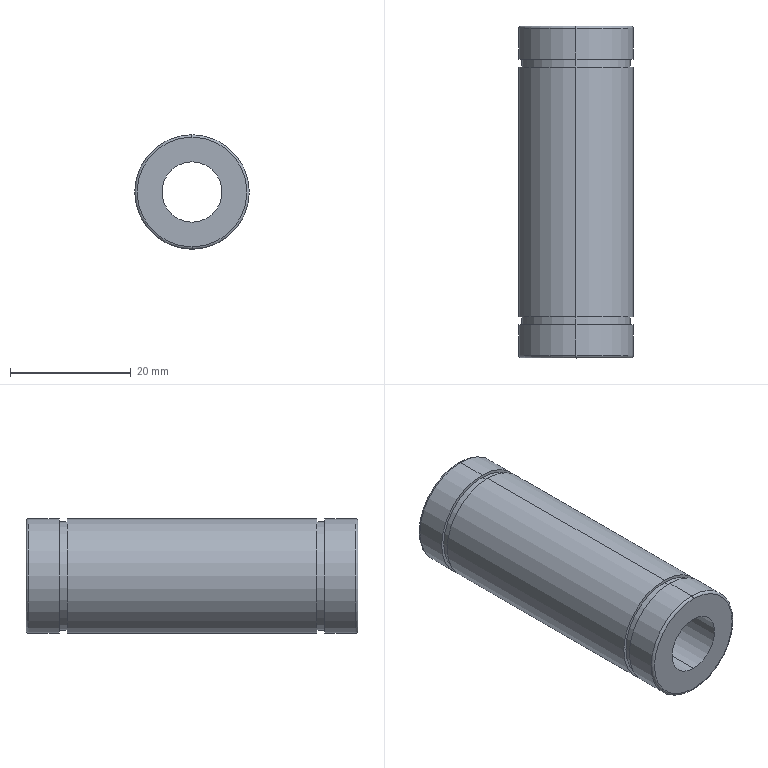Component | SolidWorks | LMUW10-3 | 1 solid | 22 faces | box 19 x 55 x 19 mm | volume 11195 mm3 | cylinder 12 | plane 6 | torus 4 | commonest cylinder face diameters 19 x6 18 x4 10 x2
build123d program:
from build123d import *


with BuildPart() as part:
    # Sketch1 → Revolve1 (revolve)
    with BuildSketch(Plane.XY, mode=Mode.PRIVATE) as revolve1_sk:
        with BuildLine():
            Line((0, 9.1), (0, 5))
            Line((0, 5), (55, 5))
            Line((55, 5), (55, 9.1))
            ThreePointArc((55, 9.1), (54.883, 9.383), (54.6, 9.5))
            Line((54.6, 9.5), (49.5, 9.5))
            Line((49.5, 9.5), (49.5, 9))
            Line((49.5, 9), (48.2, 9))
            Line((48.2, 9), (48.2, 9.5))
            Line((48.2, 9.5), (6.8, 9.5))
            Line((6.8, 9.5), (6.8, 9))
            Line((6.8, 9), (5.5, 9))
            Line((5.5, 9), (5.5, 9.5))
            Line((5.5, 9.5), (0.4, 9.5))
            ThreePointArc((0.4, 9.5), (0.1172, 9.383), (0, 9.1))
        make_face()
    revolve(revolve1_sk.sketch.rotate(Axis((27.5, 0, 0), (-1, 0, 0)), 270), axis=Axis((27.5, 0, 0), (-1, 0, 0)))


solid = part.part

# Placed as in the assembly
solid = solid.moved(Location((294.5, -645.807, -22.94), (0, 0, 90)))
STEP:
#1=COLOUR_RGB('',0.7922,0.8196,0.9333);
#2=FILL_AREA_STYLE_COLOUR('',#1);
#3=FILL_AREA_STYLE('',(#2));
#4=SURFACE_STYLE_FILL_AREA(#3);
#5=SURFACE_SIDE_STYLE('',(#4));
#6=SURFACE_STYLE_USAGE(.BOTH.,#5);
#7=PRESENTATION_STYLE_ASSIGNMENT((#6));
#8=CARTESIAN_POINT('',(11.594,-25.209,-0.5292));
#9=VERTEX_POINT('',#8);
#10=CARTESIAN_POINT('',(11.594,-25.209,-1.277));
#11=VERTEX_POINT('',#10);
#12=CARTESIAN_POINT('',(11.594,-25.209,-0.9032));
#13=DIRECTION('',(0.,-1.,-0.));
#14=DIRECTION('',(-0.,0.,1.));
#15=AXIS2_PLACEMENT_3D('',#12,#13,#14);
#16=CIRCLE('',#15,0.374);
#17=EDGE_CURVE('',#9,#11,#16,.T.);
#18=ORIENTED_EDGE('',*,*,#17,.T.);
#19=CARTESIAN_POINT('',(11.594,-25.41,-1.277));
#20=VERTEX_POINT('',#19);
#21=CARTESIAN_POINT('',(11.594,-24.343,-1.277));
#22=DIRECTION('',(0.,-1.,-0.));
#23=VECTOR('',#22,39.37);
#24=LINE('',#21,#23);
#25=EDGE_CURVE('',#11,#20,#24,.T.);
#26=ORIENTED_EDGE('',*,*,#25,.T.);
#27=CARTESIAN_POINT('',(11.594,-25.41,-0.5292));
#28=VERTEX_POINT('',#27);
#29=CARTESIAN_POINT('',(11.594,-25.41,-0.9032));
#30=DIRECTION('',(0.,-1.,-0.));
#31=DIRECTION('',(-0.,0.,1.));
#32=AXIS2_PLACEMENT_3D('',#29,#30,#31);
#33=CIRCLE('',#32,0.374);
#34=EDGE_CURVE('',#28,#20,#33,.T.);
#35=ORIENTED_EDGE('',*,*,#34,.F.);
#36=CARTESIAN_POINT('',(11.594,-24.343,-0.5292));
#37=DIRECTION('',(0.,-1.,-0.));
#38=VECTOR('',#37,39.37);
#39=LINE('',#36,#38);
#40=EDGE_CURVE('',#9,#28,#39,.T.);
#41=ORIENTED_EDGE('',*,*,#40,.F.);
#42=EDGE_LOOP('',(#18,#26,#35,#41));
#43=FACE_OUTER_BOUND('',#42,.T.);
#44=CARTESIAN_POINT('',(11.594,-24.343,-0.9032));
#45=DIRECTION('',(0.,-1.,-0.));
#46=DIRECTION('',(-0.,0.,1.));
#47=AXIS2_PLACEMENT_3D('',#44,#45,#46);
#48=CYLINDRICAL_SURFACE('',#47,0.374);
#49=ADVANCED_FACE('',(#43),#48,.T.);
#50=CARTESIAN_POINT('',(11.594,-25.158,-0.5488));
#51=VERTEX_POINT('',#50);
#52=CARTESIAN_POINT('',(11.594,-25.158,-1.257));
#53=VERTEX_POINT('',#52);
#54=CARTESIAN_POINT('',(11.594,-25.158,-0.9032));
#55=DIRECTION('',(0.,-1.,-0.));
#56=DIRECTION('',(-0.,0.,1.));
#57=AXIS2_PLACEMENT_3D('',#54,#55,#56);
#58=CIRCLE('',#57,0.3543);
#59=EDGE_CURVE('',#51,#53,#58,.T.);
#60=ORIENTED_EDGE('',*,*,#59,.T.);
#61=CARTESIAN_POINT('',(11.594,-25.209,-1.257));
#62=VERTEX_POINT('',#61);
#63=CARTESIAN_POINT('',(11.594,-24.343,-1.257));
#64=DIRECTION('',(0.,-1.,-0.));
#65=VECTOR('',#64,39.37);
#66=LINE('',#63,#65);
#67=EDGE_CURVE('',#53,#62,#66,.T.);
#68=ORIENTED_EDGE('',*,*,#67,.T.);
#69=CARTESIAN_POINT('',(11.594,-25.209,-0.5488));
#70=VERTEX_POINT('',#69);
#71=CARTESIAN_POINT('',(11.594,-25.209,-0.9032));
#72=DIRECTION('',(0.,-1.,-0.));
#73=DIRECTION('',(-0.,0.,1.));
#74=AXIS2_PLACEMENT_3D('',#71,#72,#73);
#75=CIRCLE('',#74,0.3543);
#76=EDGE_CURVE('',#70,#62,#75,.T.);
#77=ORIENTED_EDGE('',*,*,#76,.F.);
#78=CARTESIAN_POINT('',(11.594,-24.343,-0.5488));
#79=DIRECTION('',(0.,-1.,-0.));
#80=VECTOR('',#79,39.37);
#81=LINE('',#78,#80);
#82=EDGE_CURVE('',#51,#70,#81,.T.);
#83=ORIENTED_EDGE('',*,*,#82,.F.);
#84=EDGE_LOOP('',(#60,#68,#77,#83));
#85=FACE_OUTER_BOUND('',#84,.T.);
#86=CARTESIAN_POINT('',(11.594,-24.343,-0.9032));
#87=DIRECTION('',(0.,-1.,-0.));
#88=DIRECTION('',(-0.,0.,1.));
#89=AXIS2_PLACEMENT_3D('',#86,#87,#88);
#90=CYLINDRICAL_SURFACE('',#89,0.3543);
#91=ADVANCED_FACE('',(#85),#90,.T.);
#92=CARTESIAN_POINT('',(11.594,-23.528,-0.5292));
#93=VERTEX_POINT('',#92);
#94=CARTESIAN_POINT('',(11.594,-23.528,-1.277));
#95=VERTEX_POINT('',#94);
#96=CARTESIAN_POINT('',(11.594,-23.528,-0.9032));
#97=DIRECTION('',(0.,-1.,-0.));
#98=DIRECTION('',(-0.,0.,1.));
#99=AXIS2_PLACEMENT_3D('',#96,#97,#98);
#100=CIRCLE('',#99,0.374);
#101=EDGE_CURVE('',#93,#95,#100,.T.);
#102=ORIENTED_EDGE('',*,*,#101,.T.);
#103=CARTESIAN_POINT('',(11.594,-25.158,-1.277));
#104=VERTEX_POINT('',#103);
#105=CARTESIAN_POINT('',(11.594,-24.343,-1.277));
#106=DIRECTION('',(0.,-1.,-0.));
#107=VECTOR('',#106,39.37);
#108=LINE('',#105,#107);
#109=EDGE_CURVE('',#95,#104,#108,.T.);
#110=ORIENTED_EDGE('',*,*,#109,.T.);
#111=CARTESIAN_POINT('',(11.594,-25.158,-0.5292));
#112=VERTEX_POINT('',#111);
#113=CARTESIAN_POINT('',(11.594,-25.158,-0.9032));
#114=DIRECTION('',(0.,-1.,-0.));
#115=DIRECTION('',(-0.,0.,1.));
#116=AXIS2_PLACEMENT_3D('',#113,#114,#115);
#117=CIRCLE('',#116,0.374);
#118=EDGE_CURVE('',#112,#104,#117,.T.);
#119=ORIENTED_EDGE('',*,*,#118,.F.);
#120=CARTESIAN_POINT('',(11.594,-24.343,-0.5292));
#121=DIRECTION('',(0.,-1.,-0.));
#122=VECTOR('',#121,39.37);
#123=LINE('',#120,#122);
#124=EDGE_CURVE('',#93,#112,#123,.T.);
#125=ORIENTED_EDGE('',*,*,#124,.F.);
#126=EDGE_LOOP('',(#102,#110,#119,#125));
#127=FACE_OUTER_BOUND('',#126,.T.);
#128=CARTESIAN_POINT('',(11.594,-24.343,-0.9032));
#129=DIRECTION('',(0.,-1.,-0.));
#130=DIRECTION('',(-0.,0.,1.));
#131=AXIS2_PLACEMENT_3D('',#128,#129,#130);
#132=CYLINDRICAL_SURFACE('',#131,0.374);
#133=ADVANCED_FACE('',(#127),#132,.T.);
#134=CARTESIAN_POINT('',(11.594,-23.477,-0.5488));
#135=VERTEX_POINT('',#134);
#136=CARTESIAN_POINT('',(11.594,-23.477,-1.257));
#137=VERTEX_POINT('',#136);
#138=CARTESIAN_POINT('',(11.594,-23.477,-0.9032));
#139=DIRECTION('',(0.,-1.,-0.));
#140=DIRECTION('',(-0.,0.,1.));
#141=AXIS2_PLACEMENT_3D('',#138,#139,#140);
#142=CIRCLE('',#141,0.3543);
#143=EDGE_CURVE('',#135,#137,#142,.T.);
#144=ORIENTED_EDGE('',*,*,#143,.T.);
#145=CARTESIAN_POINT('',(11.594,-23.528,-1.257));
#146=VERTEX_POINT('',#145);
#147=CARTESIAN_POINT('',(11.594,-24.343,-1.257));
#148=DIRECTION('',(0.,-1.,-0.));
#149=VECTOR('',#148,39.37);
#150=LINE('',#147,#149);
#151=EDGE_CURVE('',#137,#146,#150,.T.);
#152=ORIENTED_EDGE('',*,*,#151,.T.);
#153=CARTESIAN_POINT('',(11.594,-23.528,-0.5488));
#154=VERTEX_POINT('',#153);
#155=CARTESIAN_POINT('',(11.594,-23.528,-0.9032));
#156=DIRECTION('',(0.,-1.,-0.));
#157=DIRECTION('',(-0.,0.,1.));
#158=AXIS2_PLACEMENT_3D('',#155,#156,#157);
#159=CIRCLE('',#158,0.3543);
#160=EDGE_CURVE('',#154,#146,#159,.T.);
#161=ORIENTED_EDGE('',*,*,#160,.F.);
#162=CARTESIAN_POINT('',(11.594,-24.343,-0.5488));
#163=DIRECTION('',(0.,-1.,-0.));
#164=VECTOR('',#163,39.37);
#165=LINE('',#162,#164);
#166=EDGE_CURVE('',#135,#154,#165,.T.);
#167=ORIENTED_EDGE('',*,*,#166,.F.);
#168=EDGE_LOOP('',(#144,#152,#161,#167));
#169=FACE_OUTER_BOUND('',#168,.T.);
#170=CARTESIAN_POINT('',(11.594,-24.343,-0.9032));
#171=DIRECTION('',(0.,-1.,-0.));
#172=DIRECTION('',(-0.,0.,1.));
#173=AXIS2_PLACEMENT_3D('',#170,#171,#172);
#174=CYLINDRICAL_SURFACE('',#173,0.3543);
#175=ADVANCED_FACE('',(#169),#174,.T.);
#176=CARTESIAN_POINT('',(11.594,-23.276,-0.5292));
#177=VERTEX_POINT('',#176);
#178=CARTESIAN_POINT('',(11.594,-23.276,-1.277));
#179=VERTEX_POINT('',#178);
#180=CARTESIAN_POINT('',(11.594,-23.276,-0.9032));
#181=DIRECTION('',(0.,-1.,-0.));
#182=DIRECTION('',(-0.,0.,1.));
#183=AXIS2_PLACEMENT_3D('',#180,#181,#182);
#184=CIRCLE('',#183,0.374);
#185=EDGE_CURVE('',#177,#179,#184,.T.);
#186=ORIENTED_EDGE('',*,*,#185,.T.);
#187=CARTESIAN_POINT('',(11.594,-23.477,-1.277));
#188=VERTEX_POINT('',#187);
#189=CARTESIAN_POINT('',(11.594,-24.343,-1.277));
#190=DIRECTION('',(0.,-1.,-0.));
#191=VECTOR('',#190,39.37);
#192=LINE('',#189,#191);
#193=EDGE_CURVE('',#179,#188,#192,.T.);
#194=ORIENTED_EDGE('',*,*,#193,.T.);
#195=CARTESIAN_POINT('',(11.594,-23.477,-0.5292));
#196=VERTEX_POINT('',#195);
#197=CARTESIAN_POINT('',(11.594,-23.477,-0.9032));
#198=DIRECTION('',(0.,-1.,-0.));
#199=DIRECTION('',(-0.,0.,1.));
#200=AXIS2_PLACEMENT_3D('',#197,#198,#199);
#201=CIRCLE('',#200,0.374);
#202=EDGE_CURVE('',#196,#188,#201,.T.);
#203=ORIENTED_EDGE('',*,*,#202,.F.);
#204=CARTESIAN_POINT('',(11.594,-24.343,-0.5292));
#205=DIRECTION('',(0.,-1.,-0.));
#206=VECTOR('',#205,39.37);
#207=LINE('',#204,#206);
#208=EDGE_CURVE('',#177,#196,#207,.T.);
#209=ORIENTED_EDGE('',*,*,#208,.F.);
#210=EDGE_LOOP('',(#186,#194,#203,#209));
#211=FACE_OUTER_BOUND('',#210,.T.);
#212=CARTESIAN_POINT('',(11.594,-24.343,-0.9032));
#213=DIRECTION('',(0.,-1.,-0.));
#214=DIRECTION('',(-0.,0.,1.));
#215=AXIS2_PLACEMENT_3D('',#212,#213,#214);
#216=CYLINDRICAL_SURFACE('',#215,0.374);
#217=ADVANCED_FACE('',(#211),#216,.T.);
#218=CARTESIAN_POINT('',(11.594,-23.26,-0.5449));
#219=VERTEX_POINT('',#218);
#220=CARTESIAN_POINT('',(11.594,-23.26,-1.261));
#221=VERTEX_POINT('',#220);
#222=CARTESIAN_POINT('',(11.594,-23.26,-0.9032));
#223=DIRECTION('',(0.,-1.,-0.));
#224=DIRECTION('',(-0.,0.,1.));
#225=AXIS2_PLACEMENT_3D('',#222,#223,#224);
#226=CIRCLE('',#225,0.3583);
#227=EDGE_CURVE('',#219,#221,#226,.T.);
#228=ORIENTED_EDGE('',*,*,#227,.T.);
#229=CARTESIAN_POINT('',(11.594,-23.276,-1.261));
#230=DIRECTION('',(-1.,-0.,-0.));
#231=DIRECTION('',(0.,0.,1.));
#232=AXIS2_PLACEMENT_3D('',#229,#230,#231);
#233=CIRCLE('',#232,0.01575);
#234=EDGE_CURVE('',#221,#179,#233,.T.);
#235=ORIENTED_EDGE('',*,*,#234,.T.);
#236=ORIENTED_EDGE('',*,*,#185,.F.);
#237=CARTESIAN_POINT('',(11.594,-23.276,-0.5449));
#238=DIRECTION('',(1.,0.,0.));
#239=DIRECTION('',(0.,0.,-1.));
#240=AXIS2_PLACEMENT_3D('',#237,#238,#239);
#241=CIRCLE('',#240,0.01575);
#242=EDGE_CURVE('',#219,#177,#241,.T.);
#243=ORIENTED_EDGE('',*,*,#242,.F.);
#244=EDGE_LOOP('',(#228,#235,#236,#243));
#245=FACE_OUTER_BOUND('',#244,.T.);
#246=CARTESIAN_POINT('',(11.594,-23.276,-0.9032));
#247=DIRECTION('',(0.,-1.,-0.));
#248=DIRECTION('',(-0.,-0.,1.));
#249=AXIS2_PLACEMENT_3D('',#246,#247,#248);
#250=TOROIDAL_SURFACE('',#249,0.3583,0.01575);
#251=ADVANCED_FACE('',(#245),#250,.T.);
#252=CARTESIAN_POINT('',(11.594,-23.26,-1.1));
#253=VERTEX_POINT('',#252);
#254=CARTESIAN_POINT('',(11.594,-23.26,-0.7063));
#255=VERTEX_POINT('',#254);
#256=CARTESIAN_POINT('',(11.594,-23.26,-0.9032));
#257=DIRECTION('',(0.,-1.,-0.));
#258=DIRECTION('',(-0.,0.,1.));
#259=AXIS2_PLACEMENT_3D('',#256,#257,#258);
#260=CIRCLE('',#259,0.1969);
#261=EDGE_CURVE('',#253,#255,#260,.T.);
#262=ORIENTED_EDGE('',*,*,#261,.F.);
#263=CARTESIAN_POINT('',(11.594,-25.425,-1.1));
#264=VERTEX_POINT('',#263);
#265=CARTESIAN_POINT('',(11.594,-24.343,-1.1));
#266=DIRECTION('',(0.,-1.,-0.));
#267=VECTOR('',#266,39.37);
#268=LINE('',#265,#267);
#269=EDGE_CURVE('',#253,#264,#268,.T.);
#270=ORIENTED_EDGE('',*,*,#269,.T.);
#271=CARTESIAN_POINT('',(11.594,-25.425,-0.7063));
#272=VERTEX_POINT('',#271);
#273=CARTESIAN_POINT('',(11.594,-25.425,-0.9032));
#274=DIRECTION('',(0.,-1.,-0.));
#275=DIRECTION('',(-0.,0.,1.));
#276=AXIS2_PLACEMENT_3D('',#273,#274,#275);
#277=CIRCLE('',#276,0.1969);
#278=EDGE_CURVE('',#264,#272,#277,.T.);
#279=ORIENTED_EDGE('',*,*,#278,.T.);
#280=CARTESIAN_POINT('',(11.594,-24.343,-0.7063));
#281=DIRECTION('',(0.,-1.,-0.));
#282=VECTOR('',#281,39.37);
#283=LINE('',#280,#282);
#284=EDGE_CURVE('',#255,#272,#283,.T.);
#285=ORIENTED_EDGE('',*,*,#284,.F.);
#286=EDGE_LOOP('',(#262,#270,#279,#285));
#287=FACE_OUTER_BOUND('',#286,.T.);
#288=CARTESIAN_POINT('',(11.594,-24.343,-0.9032));
#289=DIRECTION('',(0.,-1.,-0.));
#290=DIRECTION('',(-0.,0.,1.));
#291=AXIS2_PLACEMENT_3D('',#288,#289,#290);
#292=CYLINDRICAL_SURFACE('',#291,0.1969);
#293=ADVANCED_FACE('',(#287),#292,.F.);
#294=ORIENTED_EDGE('',*,*,#34,.T.);
#295=CARTESIAN_POINT('',(11.594,-25.425,-1.261));
#296=VERTEX_POINT('',#295);
#297=CARTESIAN_POINT('',(11.594,-25.41,-1.261));
#298=DIRECTION('',(-1.,-0.,-0.));
#299=DIRECTION('',(0.,0.,1.));
#300=AXIS2_PLACEMENT_3D('',#297,#298,#299);
#301=CIRCLE('',#300,0.01575);
#302=EDGE_CURVE('',#20,#296,#301,.T.);
#303=ORIENTED_EDGE('',*,*,#302,.T.);
#304=CARTESIAN_POINT('',(11.594,-25.425,-0.5449));
#305=VERTEX_POINT('',#304);
#306=CARTESIAN_POINT('',(11.594,-25.425,-0.9032));
#307=DIRECTION('',(0.,-1.,-0.));
#308=DIRECTION('',(-0.,0.,1.));
#309=AXIS2_PLACEMENT_3D('',#306,#307,#308);
#310=CIRCLE('',#309,0.3583);
#311=EDGE_CURVE('',#305,#296,#310,.T.);
#312=ORIENTED_EDGE('',*,*,#311,.F.);
#313=CARTESIAN_POINT('',(11.594,-25.41,-0.5449));
#314=DIRECTION('',(1.,0.,0.));
#315=DIRECTION('',(0.,0.,-1.));
#316=AXIS2_PLACEMENT_3D('',#313,#314,#315);
#317=CIRCLE('',#316,0.01575);
#318=EDGE_CURVE('',#28,#305,#317,.T.);
#319=ORIENTED_EDGE('',*,*,#318,.F.);
#320=EDGE_LOOP('',(#294,#303,#312,#319));
#321=FACE_OUTER_BOUND('',#320,.T.);
#322=CARTESIAN_POINT('',(11.594,-25.41,-0.9032));
#323=DIRECTION('',(0.,-1.,-0.));
#324=DIRECTION('',(-0.,-0.,1.));
#325=AXIS2_PLACEMENT_3D('',#322,#323,#324);
#326=TOROIDAL_SURFACE('',#325,0.3583,0.01575);
#327=ADVANCED_FACE('',(#321),#326,.T.);
#328=ORIENTED_EDGE('',*,*,#302,.F.);
#329=CARTESIAN_POINT('',(11.594,-25.41,-0.9032));
#330=DIRECTION('',(0.,-1.,-0.));
#331=DIRECTION('',(-0.,0.,1.));
#332=AXIS2_PLACEMENT_3D('',#329,#330,#331);
#333=CIRCLE('',#332,0.374);
#334=EDGE_CURVE('',#20,#28,#333,.T.);
#335=ORIENTED_EDGE('',*,*,#334,.T.);
#336=ORIENTED_EDGE('',*,*,#318,.T.);
#337=CARTESIAN_POINT('',(11.594,-25.425,-0.9032));
#338=DIRECTION('',(0.,-1.,-0.));
#339=DIRECTION('',(-0.,0.,1.));
#340=AXIS2_PLACEMENT_3D('',#337,#338,#339);
#341=CIRCLE('',#340,0.3583);
#342=EDGE_CURVE('',#296,#305,#341,.T.);
#343=ORIENTED_EDGE('',*,*,#342,.F.);
#344=EDGE_LOOP('',(#328,#335,#336,#343));
#345=FACE_OUTER_BOUND('',#344,.T.);
#346=CARTESIAN_POINT('',(11.594,-25.41,-0.9032));
#347=DIRECTION('',(0.,-1.,-0.));
#348=DIRECTION('',(-0.,-0.,1.));
#349=AXIS2_PLACEMENT_3D('',#346,#347,#348);
#350=TOROIDAL_SURFACE('',#349,0.3583,0.01575);
#351=ADVANCED_FACE('',(#345),#350,.T.);
#352=CARTESIAN_POINT('',(11.594,-25.425,-0.9032));
#353=DIRECTION('',(0.,-1.,-0.));
#354=DIRECTION('',(-0.,0.,1.));
#355=AXIS2_PLACEMENT_3D('',#352,#353,#354);
#356=CIRCLE('',#355,0.1969);
#357=EDGE_CURVE('',#272,#264,#356,.T.);
#358=ORIENTED_EDGE('',*,*,#357,.F.);
#359=ORIENTED_EDGE('',*,*,#278,.F.);
#360=EDGE_LOOP('',(#358,#359));
#361=FACE_BOUND('',#360,.T.);
#362=ORIENTED_EDGE('',*,*,#311,.T.);
#363=ORIENTED_EDGE('',*,*,#342,.T.);
#364=EDGE_LOOP('',(#362,#363));
#365=FACE_OUTER_BOUND('',#364,.T.);
#366=CARTESIAN_POINT('',(11.236,-25.425,-0.9032));
#367=DIRECTION('',(-0.,1.,0.));
#368=DIRECTION('',(0.,0.,-1.));
#369=AXIS2_PLACEMENT_3D('',#366,#367,#368);
#370=PLANE('',#369);
#371=ADVANCED_FACE('',(#361,#365),#370,.F.);
#372=ORIENTED_EDGE('',*,*,#269,.F.);
#373=CARTESIAN_POINT('',(11.594,-23.26,-0.9032));
#374=DIRECTION('',(0.,-1.,-0.));
#375=DIRECTION('',(-0.,0.,1.));
#376=AXIS2_PLACEMENT_3D('',#373,#374,#375);
#377=CIRCLE('',#376,0.1969);
#378=EDGE_CURVE('',#255,#253,#377,.T.);
#379=ORIENTED_EDGE('',*,*,#378,.F.);
#380=ORIENTED_EDGE('',*,*,#284,.T.);
#381=ORIENTED_EDGE('',*,*,#357,.T.);
#382=EDGE_LOOP('',(#372,#379,#380,#381));
#383=FACE_OUTER_BOUND('',#382,.T.);
#384=CARTESIAN_POINT('',(11.594,-24.343,-0.9032));
#385=DIRECTION('',(0.,-1.,-0.));
#386=DIRECTION('',(-0.,0.,1.));
#387=AXIS2_PLACEMENT_3D('',#384,#385,#386);
#388=CYLINDRICAL_SURFACE('',#387,0.1969);
#389=ADVANCED_FACE('',(#383),#388,.F.);
#390=ORIENTED_EDGE('',*,*,#227,.F.);
#391=CARTESIAN_POINT('',(11.594,-23.26,-0.9032));
#392=DIRECTION('',(0.,-1.,-0.));
#393=DIRECTION('',(-0.,0.,1.));
#394=AXIS2_PLACEMENT_3D('',#391,#392,#393);
#395=CIRCLE('',#394,0.3583);
#396=EDGE_CURVE('',#221,#219,#395,.T.);
#397=ORIENTED_EDGE('',*,*,#396,.F.);
#398=EDGE_LOOP('',(#390,#397));
#399=FACE_OUTER_BOUND('',#398,.T.);
#400=ORIENTED_EDGE('',*,*,#378,.T.);
#401=ORIENTED_EDGE('',*,*,#261,.T.);
#402=EDGE_LOOP('',(#400,#401));
#403=FACE_BOUND('',#402,.T.);
#404=CARTESIAN_POINT('',(11.398,-23.26,-0.9032));
#405=DIRECTION('',(0.,-1.,-0.));
#406=DIRECTION('',(-0.,-0.,1.));
#407=AXIS2_PLACEMENT_3D('',#404,#405,#406);
#408=PLANE('',#407);
#409=ADVANCED_FACE('',(#399,#403),#408,.F.);
#410=ORIENTED_EDGE('',*,*,#234,.F.);
#411=ORIENTED_EDGE('',*,*,#396,.T.);
#412=ORIENTED_EDGE('',*,*,#242,.T.);
#413=CARTESIAN_POINT('',(11.594,-23.276,-0.9032));
#414=DIRECTION('',(0.,-1.,-0.));
#415=DIRECTION('',(-0.,0.,1.));
#416=AXIS2_PLACEMENT_3D('',#413,#414,#415);
#417=CIRCLE('',#416,0.374);
#418=EDGE_CURVE('',#179,#177,#417,.T.);
#419=ORIENTED_EDGE('',*,*,#418,.F.);
#420=EDGE_LOOP('',(#410,#411,#412,#419));
#421=FACE_OUTER_BOUND('',#420,.T.);
#422=CARTESIAN_POINT('',(11.594,-23.276,-0.9032));
#423=DIRECTION('',(0.,-1.,-0.));
#424=DIRECTION('',(-0.,-0.,1.));
#425=AXIS2_PLACEMENT_3D('',#422,#423,#424);
#426=TOROIDAL_SURFACE('',#425,0.3583,0.01575);
#427=ADVANCED_FACE('',(#421),#426,.T.);
#428=ORIENTED_EDGE('',*,*,#193,.F.);
#429=ORIENTED_EDGE('',*,*,#418,.T.);
#430=ORIENTED_EDGE('',*,*,#208,.T.);
#431=CARTESIAN_POINT('',(11.594,-23.477,-0.9032));
#432=DIRECTION('',(0.,-1.,-0.));
#433=DIRECTION('',(-0.,0.,1.));
#434=AXIS2_PLACEMENT_3D('',#431,#432,#433);
#435=CIRCLE('',#434,0.374);
#436=EDGE_CURVE('',#188,#196,#435,.T.);
#437=ORIENTED_EDGE('',*,*,#436,.F.);
#438=EDGE_LOOP('',(#428,#429,#430,#437));
#439=FACE_OUTER_BOUND('',#438,.T.);
#440=CARTESIAN_POINT('',(11.594,-24.343,-0.9032));
#441=DIRECTION('',(0.,-1.,-0.));
#442=DIRECTION('',(-0.,0.,1.));
#443=AXIS2_PLACEMENT_3D('',#440,#441,#442);
#444=CYLINDRICAL_SURFACE('',#443,0.374);
#445=ADVANCED_FACE('',(#439),#444,.T.);
#446=ORIENTED_EDGE('',*,*,#143,.F.);
#447=CARTESIAN_POINT('',(11.594,-23.477,-0.9032));
#448=DIRECTION('',(0.,-1.,-0.));
#449=DIRECTION('',(-0.,0.,1.));
#450=AXIS2_PLACEMENT_3D('',#447,#448,#449);
#451=CIRCLE('',#450,0.3543);
#452=EDGE_CURVE('',#137,#135,#451,.T.);
#453=ORIENTED_EDGE('',*,*,#452,.F.);
#454=EDGE_LOOP('',(#446,#453));
#455=FACE_BOUND('',#454,.T.);
#456=ORIENTED_EDGE('',*,*,#202,.T.);
#457=ORIENTED_EDGE('',*,*,#436,.T.);
#458=EDGE_LOOP('',(#456,#457));
#459=FACE_OUTER_BOUND('',#458,.T.);
#460=CARTESIAN_POINT('',(11.22,-23.477,-0.9032));
#461=DIRECTION('',(-0.,1.,0.));
#462=DIRECTION('',(0.,0.,-1.));
#463=AXIS2_PLACEMENT_3D('',#460,#461,#462);
#464=PLANE('',#463);
#465=ADVANCED_FACE('',(#455,#459),#464,.F.);
#466=ORIENTED_EDGE('',*,*,#151,.F.);
#467=ORIENTED_EDGE('',*,*,#452,.T.);
#468=ORIENTED_EDGE('',*,*,#166,.T.);
#469=CARTESIAN_POINT('',(11.594,-23.528,-0.9032));
#470=DIRECTION('',(0.,-1.,-0.));
#471=DIRECTION('',(-0.,0.,1.));
#472=AXIS2_PLACEMENT_3D('',#469,#470,#471);
#473=CIRCLE('',#472,0.3543);
#474=EDGE_CURVE('',#146,#154,#473,.T.);
#475=ORIENTED_EDGE('',*,*,#474,.F.);
#476=EDGE_LOOP('',(#466,#467,#468,#475));
#477=FACE_OUTER_BOUND('',#476,.T.);
#478=CARTESIAN_POINT('',(11.594,-24.343,-0.9032));
#479=DIRECTION('',(0.,-1.,-0.));
#480=DIRECTION('',(-0.,0.,1.));
#481=AXIS2_PLACEMENT_3D('',#478,#479,#480);
#482=CYLINDRICAL_SURFACE('',#481,0.3543);
#483=ADVANCED_FACE('',(#477),#482,.T.);
#484=ORIENTED_EDGE('',*,*,#101,.F.);
#485=CARTESIAN_POINT('',(11.594,-23.528,-0.9032));
#486=DIRECTION('',(0.,-1.,-0.));
#487=DIRECTION('',(-0.,0.,1.));
#488=AXIS2_PLACEMENT_3D('',#485,#486,#487);
#489=CIRCLE('',#488,0.374);
#490=EDGE_CURVE('',#95,#93,#489,.T.);
#491=ORIENTED_EDGE('',*,*,#490,.F.);
#492=EDGE_LOOP('',(#484,#491));
#493=FACE_OUTER_BOUND('',#492,.T.);
#494=ORIENTED_EDGE('',*,*,#160,.T.);
#495=ORIENTED_EDGE('',*,*,#474,.T.);
#496=EDGE_LOOP('',(#494,#495));
#497=FACE_BOUND('',#496,.T.);
#498=CARTESIAN_POINT('',(11.24,-23.528,-0.9032));
#499=DIRECTION('',(0.,-1.,-0.));
#500=DIRECTION('',(-0.,-0.,1.));
#501=AXIS2_PLACEMENT_3D('',#498,#499,#500);
#502=PLANE('',#501);
#503=ADVANCED_FACE('',(#493,#497),#502,.F.);
#504=ORIENTED_EDGE('',*,*,#109,.F.);
#505=ORIENTED_EDGE('',*,*,#490,.T.);
#506=ORIENTED_EDGE('',*,*,#124,.T.);
#507=CARTESIAN_POINT('',(11.594,-25.158,-0.9032));
#508=DIRECTION('',(0.,-1.,-0.));
#509=DIRECTION('',(-0.,0.,1.));
#510=AXIS2_PLACEMENT_3D('',#507,#508,#509);
#511=CIRCLE('',#510,0.374);
#512=EDGE_CURVE('',#104,#112,#511,.T.);
#513=ORIENTED_EDGE('',*,*,#512,.F.);
#514=EDGE_LOOP('',(#504,#505,#506,#513));
#515=FACE_OUTER_BOUND('',#514,.T.);
#516=CARTESIAN_POINT('',(11.594,-24.343,-0.9032));
#517=DIRECTION('',(0.,-1.,-0.));
#518=DIRECTION('',(-0.,0.,1.));
#519=AXIS2_PLACEMENT_3D('',#516,#517,#518);
#520=CYLINDRICAL_SURFACE('',#519,0.374);
#521=ADVANCED_FACE('',(#515),#520,.T.);
#522=ORIENTED_EDGE('',*,*,#59,.F.);
#523=CARTESIAN_POINT('',(11.594,-25.158,-0.9032));
#524=DIRECTION('',(0.,-1.,-0.));
#525=DIRECTION('',(-0.,0.,1.));
#526=AXIS2_PLACEMENT_3D('',#523,#524,#525);
#527=CIRCLE('',#526,0.3543);
#528=EDGE_CURVE('',#53,#51,#527,.T.);
#529=ORIENTED_EDGE('',*,*,#528,.F.);
#530=EDGE_LOOP('',(#522,#529));
#531=FACE_BOUND('',#530,.T.);
#532=ORIENTED_EDGE('',*,*,#118,.T.);
#533=ORIENTED_EDGE('',*,*,#512,.T.);
#534=EDGE_LOOP('',(#532,#533));
#535=FACE_OUTER_BOUND('',#534,.T.);
#536=CARTESIAN_POINT('',(11.22,-25.158,-0.9032));
#537=DIRECTION('',(-0.,1.,0.));
#538=DIRECTION('',(0.,0.,-1.));
#539=AXIS2_PLACEMENT_3D('',#536,#537,#538);
#540=PLANE('',#539);
#541=ADVANCED_FACE('',(#531,#535),#540,.F.);
#542=ORIENTED_EDGE('',*,*,#67,.F.);
#543=ORIENTED_EDGE('',*,*,#528,.T.);
#544=ORIENTED_EDGE('',*,*,#82,.T.);
#545=CARTESIAN_POINT('',(11.594,-25.209,-0.9032));
#546=DIRECTION('',(0.,-1.,-0.));
#547=DIRECTION('',(-0.,0.,1.));
#548=AXIS2_PLACEMENT_3D('',#545,#546,#547);
#549=CIRCLE('',#548,0.3543);
#550=EDGE_CURVE('',#62,#70,#549,.T.);
#551=ORIENTED_EDGE('',*,*,#550,.F.);
#552=EDGE_LOOP('',(#542,#543,#544,#551));
#553=FACE_OUTER_BOUND('',#552,.T.);
#554=CARTESIAN_POINT('',(11.594,-24.343,-0.9032));
#555=DIRECTION('',(0.,-1.,-0.));
#556=DIRECTION('',(-0.,0.,1.));
#557=AXIS2_PLACEMENT_3D('',#554,#555,#556);
#558=CYLINDRICAL_SURFACE('',#557,0.3543);
#559=ADVANCED_FACE('',(#553),#558,.T.);
#560=ORIENTED_EDGE('',*,*,#17,.F.);
#561=CARTESIAN_POINT('',(11.594,-25.209,-0.9032));
#562=DIRECTION('',(0.,-1.,-0.));
#563=DIRECTION('',(-0.,0.,1.));
#564=AXIS2_PLACEMENT_3D('',#561,#562,#563);
#565=CIRCLE('',#564,0.374);
#566=EDGE_CURVE('',#11,#9,#565,.T.);
#567=ORIENTED_EDGE('',*,*,#566,.F.);
#568=EDGE_LOOP('',(#560,#567));
#569=FACE_OUTER_BOUND('',#568,.T.);
#570=ORIENTED_EDGE('',*,*,#76,.T.);
#571=ORIENTED_EDGE('',*,*,#550,.T.);
#572=EDGE_LOOP('',(#570,#571));
#573=FACE_BOUND('',#572,.T.);
#574=CARTESIAN_POINT('',(11.24,-25.209,-0.9032));
#575=DIRECTION('',(0.,-1.,-0.));
#576=DIRECTION('',(-0.,-0.,1.));
#577=AXIS2_PLACEMENT_3D('',#574,#575,#576);
#578=PLANE('',#577);
#579=ADVANCED_FACE('',(#569,#573),#578,.F.);
#580=ORIENTED_EDGE('',*,*,#25,.F.);
#581=ORIENTED_EDGE('',*,*,#566,.T.);
#582=ORIENTED_EDGE('',*,*,#40,.T.);
#583=ORIENTED_EDGE('',*,*,#334,.F.);
#584=EDGE_LOOP('',(#580,#581,#582,#583));
#585=FACE_OUTER_BOUND('',#584,.T.);
#586=CARTESIAN_POINT('',(11.594,-24.343,-0.9032));
#587=DIRECTION('',(0.,-1.,-0.));
#588=DIRECTION('',(-0.,0.,1.));
#589=AXIS2_PLACEMENT_3D('',#586,#587,#588);
#590=CYLINDRICAL_SURFACE('',#589,0.374);
#591=ADVANCED_FACE('',(#585),#590,.T.);
#592=CLOSED_SHELL('',(#49,#91,#133,#175,#217,#251,#293,#327,#351,#371,#389,#409,#427,#445,#465,#483,#503,#521,#541,#559,#579,#591));
#593=MANIFOLD_SOLID_BREP('',#592);
#594=STYLED_ITEM('',(#7),#593);
#595=(LENGTH_UNIT()NAMED_UNIT(*)SI_UNIT($,.METRE.));
#596=LENGTH_MEASURE_WITH_UNIT(LENGTH_MEASURE(0.0254),#595);
#597=DIMENSIONAL_EXPONENTS(1.,0.,0.,0.,0.,0.,0.);
#598=(CONVERSION_BASED_UNIT('',#596)LENGTH_UNIT()NAMED_UNIT(#597));
#599=UNCERTAINTY_MEASURE_WITH_UNIT(LENGTH_MEASURE(0.00001),#598,'','');
#600=(NAMED_UNIT(*)PLANE_ANGLE_UNIT()SI_UNIT($,.RADIAN.));
#601=(NAMED_UNIT(*)SI_UNIT($,.STERADIAN.)SOLID_ANGLE_UNIT());
#602=(GEOMETRIC_REPRESENTATION_CONTEXT(3)GLOBAL_UNCERTAINTY_ASSIGNED_CONTEXT((#599))GLOBAL_UNIT_ASSIGNED_CONTEXT((#598,#600,#601))REPRESENTATION_CONTEXT('',''));
#603=MECHANICAL_DESIGN_GEOMETRIC_PRESENTATION_REPRESENTATION('',(#594),#602);
#604=CARTESIAN_POINT('',(0.,0.,0.));
#605=DIRECTION('',(0.,0.,1.));
#606=DIRECTION('',(1.,0.,0.));
#607=AXIS2_PLACEMENT_3D('',#604,#605,#606);
#608=(LENGTH_UNIT()NAMED_UNIT(*)SI_UNIT($,.METRE.));
#609=LENGTH_MEASURE_WITH_UNIT(LENGTH_MEASURE(0.0254),#608);
#610=DIMENSIONAL_EXPONENTS(1.,0.,0.,0.,0.,0.,0.);
#611=(CONVERSION_BASED_UNIT('',#609)LENGTH_UNIT()NAMED_UNIT(#610));
#612=UNCERTAINTY_MEASURE_WITH_UNIT(LENGTH_MEASURE(0.00001),#611,'','');
#613=(NAMED_UNIT(*)PLANE_ANGLE_UNIT()SI_UNIT($,.RADIAN.));
#614=(NAMED_UNIT(*)SI_UNIT($,.STERADIAN.)SOLID_ANGLE_UNIT());
#615=(GEOMETRIC_REPRESENTATION_CONTEXT(3)GLOBAL_UNCERTAINTY_ASSIGNED_CONTEXT((#612))GLOBAL_UNIT_ASSIGNED_CONTEXT((#611,#613,#614))REPRESENTATION_CONTEXT('',''));
#616=ADVANCED_BREP_SHAPE_REPRESENTATION('',(#593,#607),#615);
#617=PRESENTATION_LAYER_ASSIGNMENT('','',(#594));